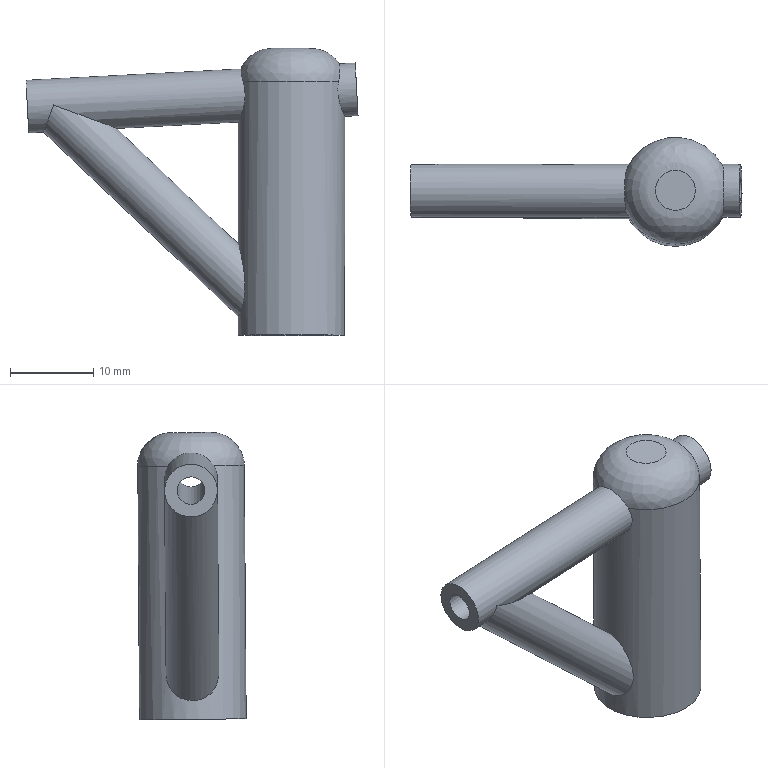Component | NX | BEARING_HOUSING | 1 solid | 16 faces | volume 3802 mm3 | cylinder 8 | plane 7 | spline 1 | commonest cylinder face diameters 6.35 x5 12.8 x1 3.3 x1 9.8 x1